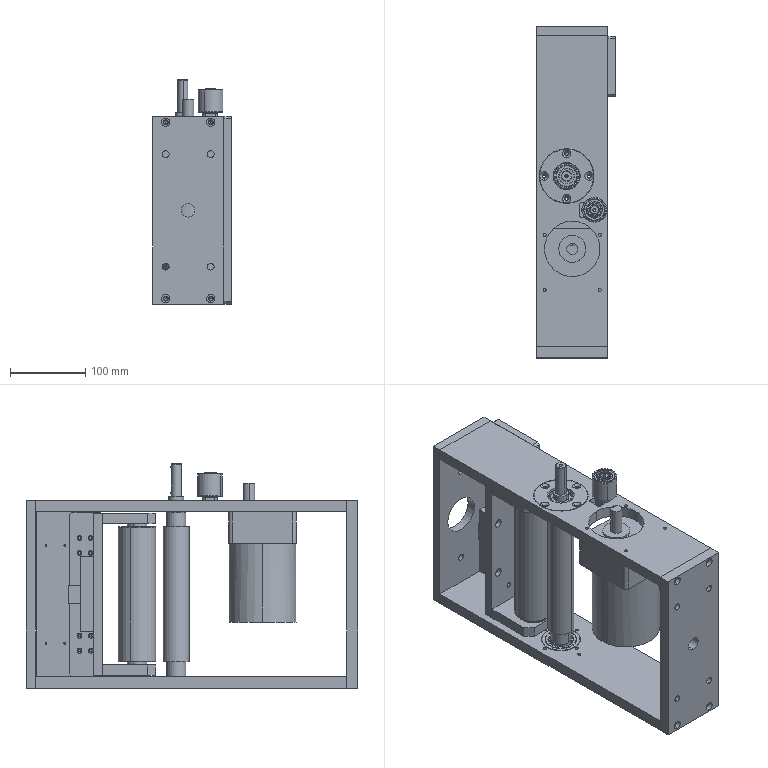Assembly | SolidWorks | mm | 25 component files | 26 solids | 1338 faces | box 105 x 442 x 299 mm | volume 3905801 mm3 | cylinder 482 | torus 338 | plane 228 | sphere 184 | cone 106 | commonest cylinder face diameters 5 x70 11 x51 6.6 x48 4.2 x30 6.5 x18 5.5 x16 42 x16 20 x16
Bill of materials:
8TC-A15004-D0-01A | 1 | #45 | Rectangular flat plate with one larger central through-hole and eight smaller through-holes in two symmetric columns.
8TC-A15004-D0-02A | 1 | #45 | Long rectangular plate with one large through-hole, one smaller through-hole with a stepped counterbore, a small rounded slot, a pattern of small holes, and holes drilled into the edges.
8TC-A15004-D0-03A | 1 | #45 | Rectangular flat plate with one large central through-hole, two medium holes on its centerline, and four small corner holes.
8TC-A15004-D0-04A | 2 | A3 | Round flanged ring: a thin circular flange with a raised cylindrical hub, a central bore with an internal step, and four equally spaced through-holes in the flange.
8TC-A15004-D0-05A | 1 | #45 | Stepped cylindrical shaft with a long main diameter and several smaller-diameter steps at each end, plus a small center hole in one end face.
8TC-A15004-D0-06A | 1 | #45 | Cylindrical body with short, smaller-diameter stepped stubs on both ends and a small center hole in one end face.
8TC-A15004-D0-07A | 2 | #45 | Thick, roughly square block with two chamfered corners on one side and an off-center circular through-bore with a stepped counterbore.
8TC-A15004-D0-08A | 1 | #45 | Rectangular thick plate with a symmetric pattern of face through-holes and a row of small holes drilled into one long edge.
8TC-A15004-D0-09A | 1 | #45 | Long rectangular plate with one large through-hole, a ring of small holes around it, and small holes drilled into the edges.
8TC-A15004-D0-10A | 1 | #45 | Thin rectangular plate with small corner chamfers, four larger corner holes and two rows of three very small holes.
8TC-A15004-D0-11A | 1 | #45 | Narrow rectangular strip plate with chamfered corners, four larger holes along one side and two groups of four small holes.
8TC-A15004-D0-13A | 1 | #45 | Rectangular block with a T-shaped (undercut) slot running along its length through one face, and four through-holes in the large face.
8TC-A15004-D0-14A | 1 | #45 | Prismatic block with a stepped, inverted-T profile: a narrower upper body on a wider base flange, with one large round through-bore through the block.
8TC-A15004-D0-15A | 1 | #45 | Turned-style part with a square base whose corners are chamfered, a short round collar on top of the base, and a taller cylindrical post with a chamfered top end and a small hole in its centre.
8TC-A15004-D0-16A | 1 | #45 | Thin-walled cylindrical sleeve or ring, open at both ends, with a small internal step or shoulder some way into the bore.
GB_CONNECTING_PIECE_RING_RRA 12 | 1 |  | Flat, open, split ring of constant thickness. A circular bore sits inside a non-concentric outer profile, with two flat lugs on either side of a straight-sided radial gap. Each lug has one small round through-hole. Shape matches an external retaining ring (circlip).
Rolling bearings 6004 GB 276-94 | 4 |  | Annular assembly shaped like an open (unshielded) radial ball bearing: an outer ring and an inner ring, coaxial and of equal width, with a single row of spherical balls between them. No visible cage or seals. The face view shows about 16 balls.
Rolling bearings 6001 GB 276-94 | 2 |  | Annular assembly shaped like an open radial ball bearing, much like the previous part: coaxial outer and inner rings of equal width with a single row of spherical balls between them. No visible cage or seals. The face view shows about 14 balls, and the bore looks slightly smaller relative to the outside diameter.
YN90G60 90JA40G15 | 1 |  | Body with a square flange: a square block with rounded corners and four corner holes sits on a cylindrical body, with a short round pilot boss and a protruding cylindrical shaft on the flange face.
Mates:
1. coincident | 8TC-A15004-D0-01A-1 face at (0, 7.5, 0) dir (0, 1, 0) | 8TC-A15004-D0-09A-1 face at (-47.5, 7.5, -110) dir (0, -1, 0)
2. width | 8TC-A15004-D0-01A-1 face at (47.5, 7.5, 125) dir (1, 0, 0) | 8TC-A15004-D0-01A-1 face at (-47.5, 7.5, 125) dir (-1, 0, 0) | 8TC-A15004-D0-09A-1 face at (47.5, 7.5, -110) dir (1, 0, 0) | 8TC-A15004-D0-09A-1 face at (-47.5, 7.5, -110) dir (-1, 0, 0)
3. coincident | 8TC-A15004-D0-01A-1 face at (-47.5, 7.5, 125) dir (0, 0, 1) | 8TC-A15004-D0-02A-2 face at (0, 215, 125) dir (0, 0, 1)
4. coincident | 8TC-A15004-D0-01A-1 face at (0, 7.5, 0) dir (0, 1, 0) | 8TC-A15004-D0-02A-2 face at (47.5, 7.5, 110) dir (0, -1, 0)
5. width | 8TC-A15004-D0-02A-2 face at (47.5, 7.5, 110) dir (1, 0, 0) | 8TC-A15004-D0-02A-2 face at (-47.5, 7.5, 110) dir (-1, 0, 0) | 8TC-A15004-D0-01A-1 face at (47.5, 7.5, 125) dir (1, 0, 0) | 8TC-A15004-D0-01A-1 face at (-47.5, 7.5, 125) dir (-1, 0, 0)
6. coincident | 8TC-A15004-D0-09A-1 face at (-47.5, 422.5, -110) dir (0, 1, 0) | 8TC-A15004-D0-03A-1 face at (0, 422.5, 0) dir (0, -1, 0)
7. width | 8TC-A15004-D0-03A-1 face at (47.5, 422.5, 125) dir (1, 0, 0) | 8TC-A15004-D0-03A-1 face at (-47.5, 422.5, 125) dir (-1, 0, 0) | 8TC-A15004-D0-09A-1 face at (47.5, 7.5, -110) dir (1, 0, 0) | 8TC-A15004-D0-09A-1 face at (-47.5, 7.5, -110) dir (-1, 0, 0)
8. coincident | 8TC-A15004-D0-09A-1 face at (0, 215, -125) dir (0, 0, -1) | 8TC-A15004-D0-03A-1 face at (-47.5, 422.5, -125) dir (0, 0, -1)
9. concentric | 8TC-A15004-D0-09A-1 face at (-7.5, 234.5, -110) dir (0, 0, -1) r 26 | 8TC-A15004-D0-04A-1 face at (-7.5, 234.5, -125) dir (0, 0, -1) r 26
10. concentric | 8TC-A15004-D0-02A-2 face at (-7.5, 234.5, 110) dir (0, 0, 1) r 26 | 8TC-A15004-D0-04A-2 face at (-7.5, 234.5, 125) dir (0, 0, 1) r 26
11. coincident | 8TC-A15004-D0-04A-1 face at (-28.5, 234.5, -122) dir (0, 0, 1) | deep groove ball bearings gb-1 face at (-7.5, 255.5, -122) dir (0, 0, -1)
12. concentric | 8TC-A15004-D0-04A-1 face at (-7.5, 234.5, -125) dir (0, 0, -1) r 21 | deep groove ball bearings gb-1 face at (-7.5, 234.5, -107.289) dir (0, 0, 1) r 21
13. concentric | 8TC-A15004-D0-04A-2 face at (-7.5, 234.5, 125) dir (0, 0, 1) r 21 | deep groove ball bearings gb-2 face at (-7.5, 234.5, 124.711) dir (0, 0, 1) r 21
14. coincident | 8TC-A15004-D0-04A-2 face at (-7.5, 213.5, 122) dir (0, 0, -1) | deep groove ball bearings gb-2 face at (-7.5, 255.5, 122) dir (0, 0, 1)
15. concentric | deep groove ball bearings gb-1 face at (-7.5, 234.5, -109.029) dir (0, 0, 1) r 10 | 8TC-A15004-D0-05A-1 face at (-7.5, 234.5, 174) dir (0, 0, 1) r 10
16. coincident | deep groove ball bearings gb-1 face at (-7.5, 248.167, -110) dir (0, 0, 1) | 8TC-A15004-D0-05A-1 face at (-8.858, 247.429, -110) dir (0, 0, -1)
17. coincident | deep groove ball bearings gb-2 face at (-7.5, 244.5, 110) dir (0, 0, -1) | 8TC-A15004-D0-05A-1 face at (-8.858, 247.429, 110) dir (0, 0, 1)
18. coincident | 8TC-A15004-D0-06A-1 face at (4.508, 281.52, 94) dir (0, 0, 1) | deep groove ball bearings gb-3 face at (-3.67, 295.737, 94) dir (0, 0, -1)
19. concentric | 8TC-A15004-D0-06A-1 face at (-7.5, 286.5, -106) dir (0, 0, -1) r 10 | deep groove ball bearings gb-3 face at (-7.5, 286.5, 106.971) dir (0, 0, 1) r 10
20. coincident | 8TC-A15004-D0-06A-1 face at (4.508, 281.52, -94) dir (0, 0, -1) | deep groove ball bearings gb-4 face at (-2.265, 299.124, -94) dir (0, 0, 1)
21. concentric | 8TC-A15004-D0-06A-1 face at (-7.5, 286.5, -106) dir (0, 0, -1) r 10 | deep groove ball bearings gb-4 face at (-7.5, 286.5, -93.029) dir (0, 0, 1) r 10
22. coincident | deep groove ball bearings gb-4 face at (0.544, 305.898, -106) dir (0, 0, -1) | 8TC-A15004-D0-07A-1 face at (-7.5, 286.5, -106) dir (0, 0, 1)
23. concentric | deep groove ball bearings gb-4 face at (-7.5, 286.5, -91.289) dir (0, 0, 1) r 21 | 8TC-A15004-D0-07A-1 face at (-7.5, 286.5, -106) dir (0, 0, 1) r 21
24. coincident | deep groove ball bearings gb-3 face at (0.544, 305.898, 106) dir (0, 0, 1) | 8TC-A15004-D0-07A-2 face at (-7.5, 286.5, 106) dir (0, 0, -1)
25. concentric | deep groove ball bearings gb-3 face at (-7.5, 286.5, 108.711) dir (0, 0, 1) r 21 | 8TC-A15004-D0-07A-2 face at (-7.5, 286.5, 106) dir (0, 0, -1) r 21
26. coincident | 8TC-A15004-D0-07A-1 face at (-39.5, 332.5, -94) dir (0, 1, 0) | 8TC-A15004-D0-07A-2 face at (24.5, 332.5, 94) dir (0, 1, 0)
27. coincident | 8TC-A15004-D0-07A-2 face at (24.5, 332.5, 94) dir (0, 1, 0) | 8TC-A15004-D0-08A-1 face at (-7.5, 332.5, 0) dir (0, -1, 0)
28. coincident | 8TC-A15004-D0-07A-2 face at (-7.5, 297.5, 108) dir (0, 0, 1) | 8TC-A15004-D0-08A-1 face at (-39.5, 332.5, 108) dir (0, 0, 1)
29. width | 8TC-A15004-D0-08A-1 face at (24.5, 332.5, 108) dir (1, 0, 0) | 8TC-A15004-D0-08A-1 face at (-39.5, 332.5, 108) dir (-1, 0, 0) | 8TC-A15004-D0-07A-2 face at (24.5, 262.5, 94) dir (1, 0, 0) | 8TC-A15004-D0-07A-2 face at (-39.5, 262.5, 94) dir (-1, 0, 0)
30. width | 8TC-A15004-D0-08A-1 face at (-39.5, 332.5, 108) dir (0, 0, 1) | 8TC-A15004-D0-08A-1 face at (-39.5, 332.5, -108) dir (0, 0, -1) | 8TC-A15004-D0-09A-1 face at (0, 215, -110) dir (0, 0, 1) | 8TC-A15004-D0-02A-2 face at (0, 215, 110) dir (0, 0, -1)
31. parallel | 8TC-A15004-D0-03A-1 face at (0, 422.5, 0) dir (0, -1, 0) | 8TC-A15004-D0-08A-1 face at (-7.5, 344.5, 0) dir (0, 1, 0)
32. width | 8TC-A15004-D0-10A-1 face at (47.5, 420.5, 125) dir (0, 0, 1) | 8TC-A15004-D0-10A-1 face at (47.5, 420.5, -125) dir (0, 0, -1) | 8TC-A15004-D0-09A-1 face at (0, 215, -125) dir (0, 0, -1) | 8TC-A15004-D0-02A-2 face at (0, 215, 125) dir (0, 0, 1)
33. distance | 8TC-A15004-D0-02A-2 face at (47.5, 422.5, 110) dir (0, 1, 0) | 8TC-A15004-D0-10A-1 face at (47.5, 420.5, -125) dir (0, 1, 0)
34. width | 8TC-A15004-D0-11A-1 face at (24.5, 376.5, -109) dir (0, 0, -1) | 8TC-A15004-D0-11A-1 face at (24.5, 376.5, 109) dir (0, 0, 1) | 8TC-A15004-D0-08A-1 face at (-39.5, 332.5, 108) dir (0, 0, 1) | 8TC-A15004-D0-08A-1 face at (-39.5, 332.5, -108) dir (0, 0, -1)
35. coincident | 8TC-A15004-D0-09A-1 face at (47.5, 7.5, -110) dir (1, 0, 0) | 8TC-A15004-D0-10A-1 face at (47.5, 380.5, 0) dir (-1, 0, 0)
36. coincident | 8TC-A15004-D0-07A-2 face at (24.5, 262.5, 94) dir (1, 0, 0) | 8TC-A15004-D0-11A-1 face at (24.5, 354.5, 0) dir (-1, 0, 0)
37. coincident | 8TC-A15004-D0-02A-2 face at (-7.5, 234.5, 120) dir (0, 0, 1) | 8TC-A15004-D0-04A-2 face at (-7.5, 198.5, 120) dir (0, 0, -1)
38. coincident | 8TC-A15004-D0-09A-1 face at (-7.5, 234.5, -120) dir (0, 0, -1) | 8TC-A15004-D0-04A-1 face at (-43.5, 234.5, -120) dir (0, 0, 1)
39. coincident | 8TC-A15004-D0-08A-1 face at (-7.5, 344.5, 0) dir (0, 1, 0) | 8TC-A15004-D0-13A-2 face at (-7.5, 344.5, 0) dir (0, -1, 0)
40. width | 8TC-A15004-D0-08A-1 face at (-39.5, 332.5, 108) dir (-1, 0, 0) | 8TC-A15004-D0-08A-1 face at (24.5, 332.5, 108) dir (1, 0, 0) | 8TC-A15004-D0-13A-2 face at (17.5, 362.5, 50) dir (1, 0, 0) | 8TC-A15004-D0-13A-2 face at (-32.5, 362.5, 50) dir (-1, 0, 0)
41. width | 8TC-A15004-D0-08A-1 face at (-39.5, 332.5, 108) dir (0, 0, 1) | 8TC-A15004-D0-08A-1 face at (-39.5, 332.5, -108) dir (0, 0, -1) | 8TC-A15004-D0-13A-2 face at (17.5, 362.5, 50) dir (0, 0, 1) | 8TC-A15004-D0-13A-2 face at (17.5, 362.5, -50) dir (0, 0, -1)
42. coincident | 8TC-A15004-D0-13A-2 face at (8.5, 353, 50) dir (0, 1, 0) | 8TC-A15004-D0-14A-1 face at (-7.5, 353, 0) dir (0, -1, 0)
43. width | 8TC-A15004-D0-14A-1 face at (8, 378, -12.5) dir (1, 0, 0) | 8TC-A15004-D0-14A-1 face at (-23, 378, -12.5) dir (-1, 0, 0) | 8TC-A15004-D0-13A-2 face at (8.5, 353, 50) dir (-1, 0, 0) | 8TC-A15004-D0-13A-2 face at (-23.5, 353, 50) dir (1, 0, 0)
44. width | 8TC-A15004-D0-13A-2 face at (17.5, 362.5, 50) dir (0, 0, 1) | 8TC-A15004-D0-13A-2 face at (17.5, 362.5, -50) dir (0, 0, -1) | 8TC-A15004-D0-14A-1 face at (-23, 378, 12.5) dir (0, 0, 1) | 8TC-A15004-D0-14A-1 face at (-23, 378, -12.5) dir (0, 0, -1)
45. concentric | 8TC-A15004-D0-09A-1 face at (-7.5, 264.5, -120) dir (0, 0, -1) r 2.1 | 8TC-A15004-D0-04A-1 face at (-7.5, 264.5, -125) dir (0, 0, -1) r 2.75
46. concentric | 8TC-A15004-D0-02A-2 face at (-7.5, 264.5, 120) dir (0, 0, 1) r 2.1 | 8TC-A15004-D0-04A-2 face at (-7.5, 264.5, 125) dir (0, 0, 1) r 2.75
47. concentric | 8TC-A15004-D0-15A-1 face at (29.5, 189.5, 116) dir (0, 0, -1) r 6 | 8TC-A15004-D0-16A-1 face at (29.5, 189.5, 161) dir (0, 0, 1) r 12
48. coincident | 8TC-A15004-D0-16A-1 face at (35.537, 199.871, 153) dir (0, 0, 1) | deep groove ball bearings gb-5 face at (29.5, 203.5, 153) dir (0, 0, -1)
49. concentric | 8TC-A15004-D0-16A-1 face at (29.5, 189.5, 161) dir (0, 0, 1) r 14 | deep groove ball bearings gb-5 face at (29.5, 189.5, 148.289) dir (0, 0, -1) r 14
50. coincident | 8TC-A15004-D0-16A-1 face at (35.537, 199.871, 139) dir (0, 0, -1) | deep groove ball bearings gb-6 face at (29.5, 203.5, 139) dir (0, 0, 1)
51. concentric | 8TC-A15004-D0-16A-1 face at (29.5, 189.5, 161) dir (0, 0, 1) r 14 | deep groove ball bearings gb-6 face at (29.5, 189.5, 126.289) dir (0, 0, -1) r 14
52. coincident | 8TC-A15004-D0-15A-1 face at (29.5, 195.5, 131) dir (0, 0, 1) | deep groove ball bearings gb-6 face at (29.5, 198.167, 131) dir (0, 0, -1)
53. coincident | 8TC-A15004-D0-02A-2 face at (0, 215, 116) dir (0, 0, 1) | 8TC-A15004-D0-15A-1 face at (29.5, 201.5, 116) dir (0, 0, -1)
54. width | 8TC-A15004-D0-15A-1 face at (19.5, 199.5, 116) dir (0, 1, 0) | 8TC-A15004-D0-15A-1 face at (19.5, 179.5, 116) dir (0, -1, 0) | 8TC-A15004-D0-02A-2 face at (36.5, 179.5, 73.944) dir (0, 1, 0) | 8TC-A15004-D0-02A-2 face at (36.5, 199.5, 73.944) dir (0, -1, 0)
55. coincident | 8TC-A15004-D0-02A-2 face at (39.5, 196.5, 73.944) dir (-1, 0, 0) | 8TC-A15004-D0-15A-1 face at (39.5, 179.5, 116) dir (1, 0, 0)
56. coincident | 8TC-A15004-D0-15A-1 face at (29.5, 195.2, 161) dir (0, 0, 1) | circlips for shaft--type a large gb-1 face at (29.5, 189.5, 161) dir (0, 0, -1)
57. coincident | 8TC-A15004-D0-08A-1 face at (-7.5, 332.5, 0) dir (0, -1, 0) | 8TC-A15004-D0-11A-1 face at (24.5, 332.5, -109) dir (0, -1, 0)
58. concentric | 8TC-A15004-D0-02A-2 face at (0, 137.5, 110) dir (0, 0, 1) r 37 | YN90G60 90JA40G15-1 face at (0, 137.5, 148) dir (0, 0, -1) r 7.5
59. coincident | 8TC-A15004-D0-02A-2 face at (0, 215, 110) dir (0, 0, -1) | YN90G60 90JA40G15-1 face at (-11422.504, 1623.724, 110) dir (0, 0, 1)